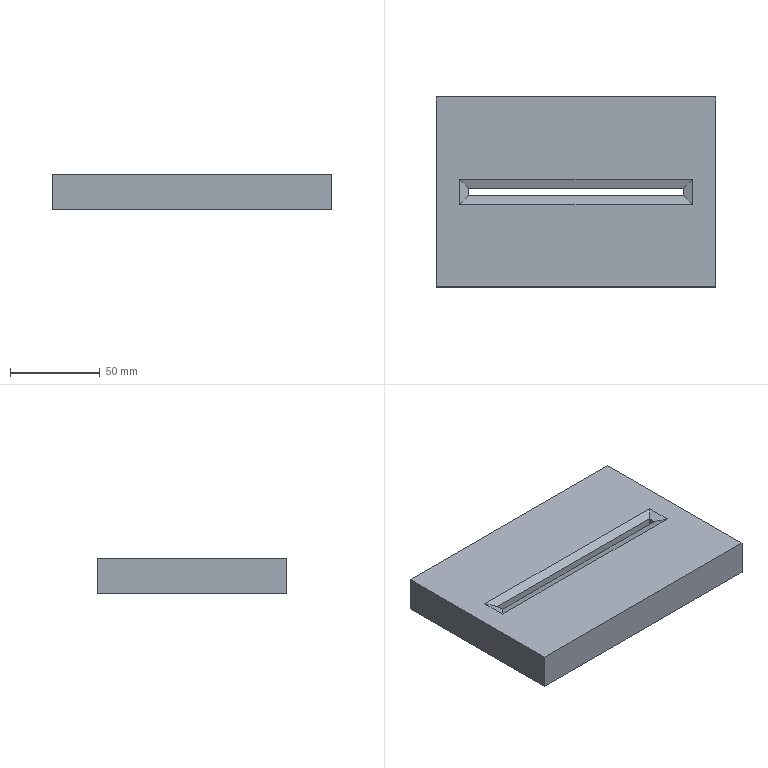Component | NX | SHE_JI-2 | 1 solid | 19 faces | volume 203771 mm3 | plane 19